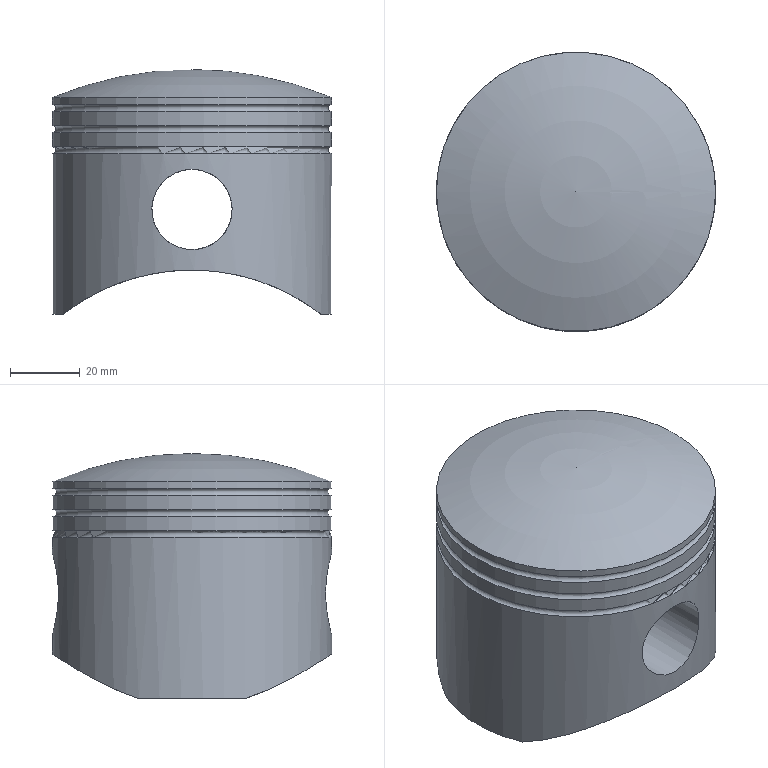Component | NX | PISTON | 1 solid | 22 faces | volume 66344 mm3 | cylinder 11 | plane 5 | torus 3 | cone 2 | sphere 1 | commonest cylinder face diameters 79.8 x4 23 x2 29 x2 120 x2 73.8 x1